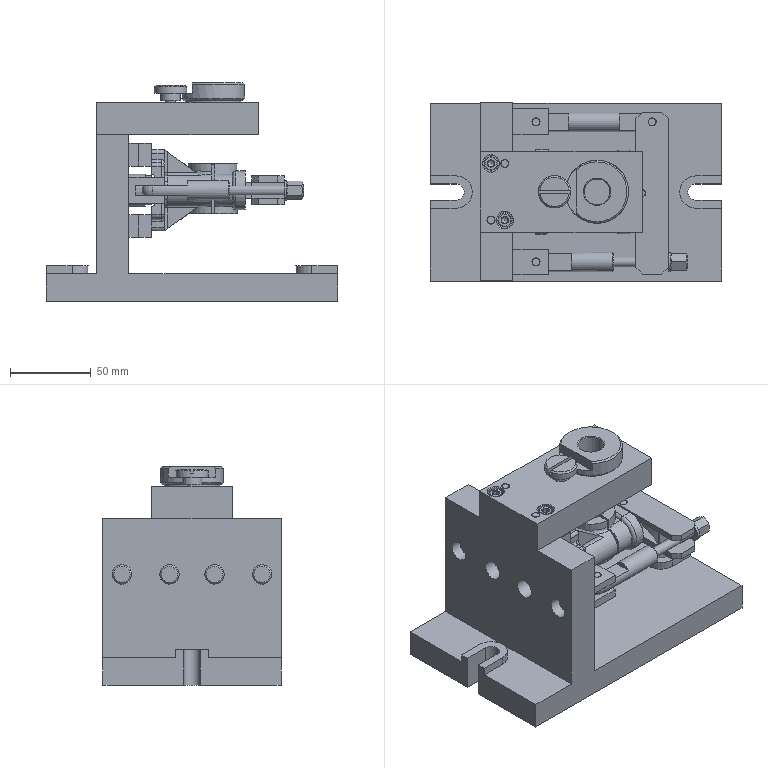Assembly | NX | mm | 30 component files | 30 solids | 587 faces | box 180 x 110 x 135 mm | volume 759036 mm3 | plane 307 | cylinder 138 | cone 108 | torus 20 | sphere 12 | spline 2 | commonest cylinder face diameters 4 x32 5 x22 10 x15 12 x12 4.826 x12 20 x8 5.5 x6 8.5 x6
Bill of materials:
unnamed part 1 | 2 |  | Stepped cylindrical pin with an integral thin collar/flange between a larger-diameter body on one side and a smaller-diameter pin on the other.
GB-T70.1-2000,M5x10 | 4 |  | Hexagon Socket Head Cap Screw, GB-T 70.1-2000,M5x10
unnamed part 2 | 1 |  | L-shaped bracket: a rectangular base plate with an upright plate at one end. The upright carries several holes, raised strips and an oblong boss with two holes.
unnamed part 3 | 2 |  | Fork-shaped (clevis-like) part: a cylindrical shank attached to a rectangular block with an open slot that forms two parallel tines, crossed by one hole.
unnamed part 4 | 1 |  | Long stepped rod with a flattened eye end that has a cross hole, a larger cylindrical collar section, a long slender shaft and a reduced-diameter end step.
GB804-1988,M6 | 1 |  | Hexagon Nut, Raised Face, GB 804-1988,M6
GB-T119.1-2000,5x16 | 2 |  | Parallel Pin, GB-T 119.1-2000,5x16
unnamed part 5 | 1 |  | Slotted-head stepped pin or shoulder-screw-like part: a large chamfered disc head with a straight slot, a shoulder, a narrow neck and a chamfered cylindrical tip.
unnamed part 6 | 1 |  | Elongated rectangular bar with clipped (chamfered) corners and an open slot at each end, giving fork-like ends. It has two small through holes.
GB-T119.1-2000,5x18 | 2 |  | Parallel Pin, GB-T 119.1-2000,5x18
unnamed part 7 | 2 |  | Rectangular block with two through holes in its largest face. Each hole has a surrounding counterbore or chamfer ring.
GB-T95-2002,M6 | 1 |  | Plain Washer, GB-T 95-2002,M6
unnamed part 8 | 1 |  | Flanged bushing: a cylindrical sleeve with a larger flange at one end. The flange has a straight flat cut on one side, and a bore runs through the full length.
GB-T119.1-2000,5x24 | 2 |  | Parallel Pin, GB-T 119.1-2000,5x24
unnamed part 9 | 1 |  | Plain cylindrical tube or ring (spacer-like sleeve) with a uniform wall and flat ends.
unnamed part 10 | 1 |  | Prismatic block with a D-shaped (circular-segment) profile: one flat side, one convex arc side and one through hole.
GB-T70.1-2000,M5x20 | 2 |  | Hexagon Socket Head Cap Screw, GB-T 70.1-2000,M5x20
unnamed part 11 | 1 |  | Thick rectangular plate with one large through hole, one smaller through hole, and two pairs of holes near one end. One hole in each pair has a counterbore-like ring.
unnamed part 12 | 1 |  | Elongated link or rod with rounded ends: a round bar with two parallel flats along its length and a full-round cylindrical middle section, with one through hole near each end.
unnamed part 13 | 1 |  | Bracket-like block with a flat rectangular flange plate at one end, a horizontal cylindrical boss running out from that flange, and a split ring clamp collar whose through-bore runs perpendicular to the boss. A slot through the ring wall splits it. The far end has an obround (rounded-slot shaped) plate with two round through-holes. Ribs or a triangular gusset join the flange to the boss, with a rectangular pocket or window framed by ribs.
Mates:
1. fix | fixture_body 1 component
2. concentric | A_locating_pin 2 edge | fixture_body 1 edge
3. concentric | A_locating_pin 1 edge | fixture_body 1 edge
4. concentric | A_support_plate 2 edge | fixture_body 1 arc
5. concentric | A_support_plate 1 edge | fixture_body 1 arc
6. concentric | connector 2 edge | fixture_body 1 edge
7. concentric | connector 1 edge | fixture_body 1 edge
8. concentric | hinge_rod 1 edge | connector 2 edge
9. concentric | screw_rod 1 edge | connector 1 edge
10. touch align | rocker_arm_shaft_seat 1 face | A_locating_pin 1 face
11. touch align | rocker_arm_shaft_seat 1 face | A_locating_pin 2 face
12. touch align | rocker_arm_shaft_seat 1 face | A_locating_pin 1 face
13. concentric | curved_clamp_block 1 edge | hinge_clamp_plate 1 edge
14. touch align | hinge_clamp_plate 1 face | hinge_rod 1 face
15. center | hinge_clamp_plate 1 face | hinge_clamp_plate 1 face | hinge_rod 1 face | hinge_rod 1 face
16. concentric | drill_jig_plate 1 edge | fixture_body 1 edge
17. concentric | bushing 1 edge | drill_jig_plate 1 edge
18. concentric | drill_bushing 1 edge | bushing 1 edge
19. touch align | drill_bushing_screw 1 face | drill_bushing 1 face
20. touch align | drill_bushing_screw 1 face | drill_jig_plate 1 face
21. concentric | GB-T70_1-2000_M5x20 2 edge | drill_jig_plate 1 edge
22. concentric | GB-T70_1-2000_M5x20 1 edge | drill_jig_plate 1 edge
23. concentric | GB-T119_1-2000_5x24 1 edge | drill_jig_plate 1 edge
24. touch align | GB-T95-2002_M6 1 face | screw_rod 1 face
25. touch align | GB-T95-2002_M6 1 face | hinge_clamp_plate 1 face
26. touch align | GB804-1988_M6 1 face | screw_rod 1 face
27. touch align | GB804-1988_M6 1 face | GB-T95-2002_M6 1 face
28. concentric | GB-T70_1-2000_M5x10 1 edge | A_support_plate 2 edge
29. concentric | GB-T70_1-2000_M5x10 2 edge | A_support_plate 2 edge
30. concentric | GB-T70_1-2000_M5x10 3 edge | A_support_plate 1 edge
31. concentric | GB-T70_1-2000_M5x10 4 edge | A_support_plate 1 edge